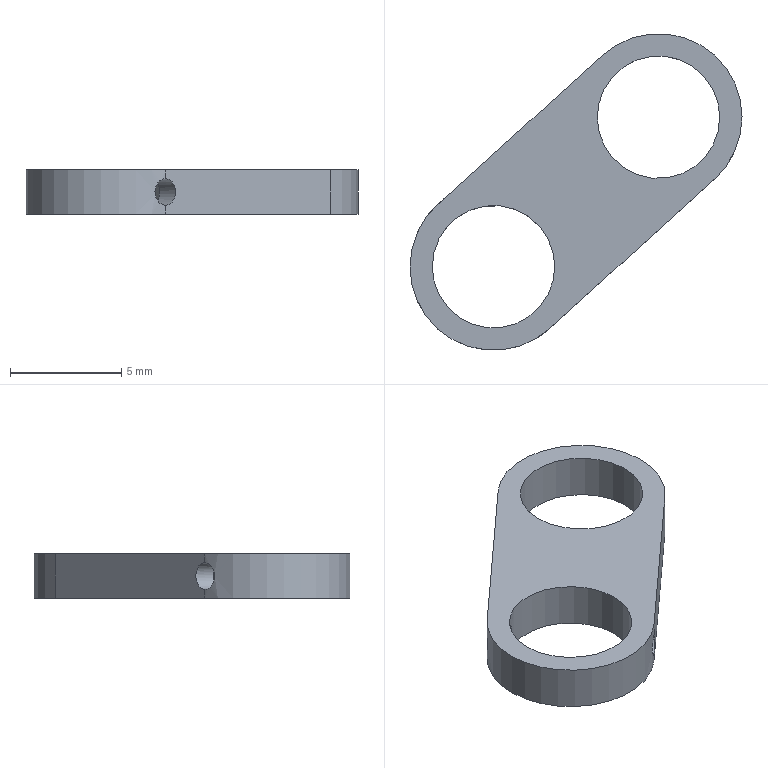Component | NX | CRANK_ROCKER_3 | 1 solid | 10 faces | volume 141 mm3 | cylinder 6 | plane 4 | commonest cylinder face diameters 7.5 x2 5.5 x2 1.2 x2